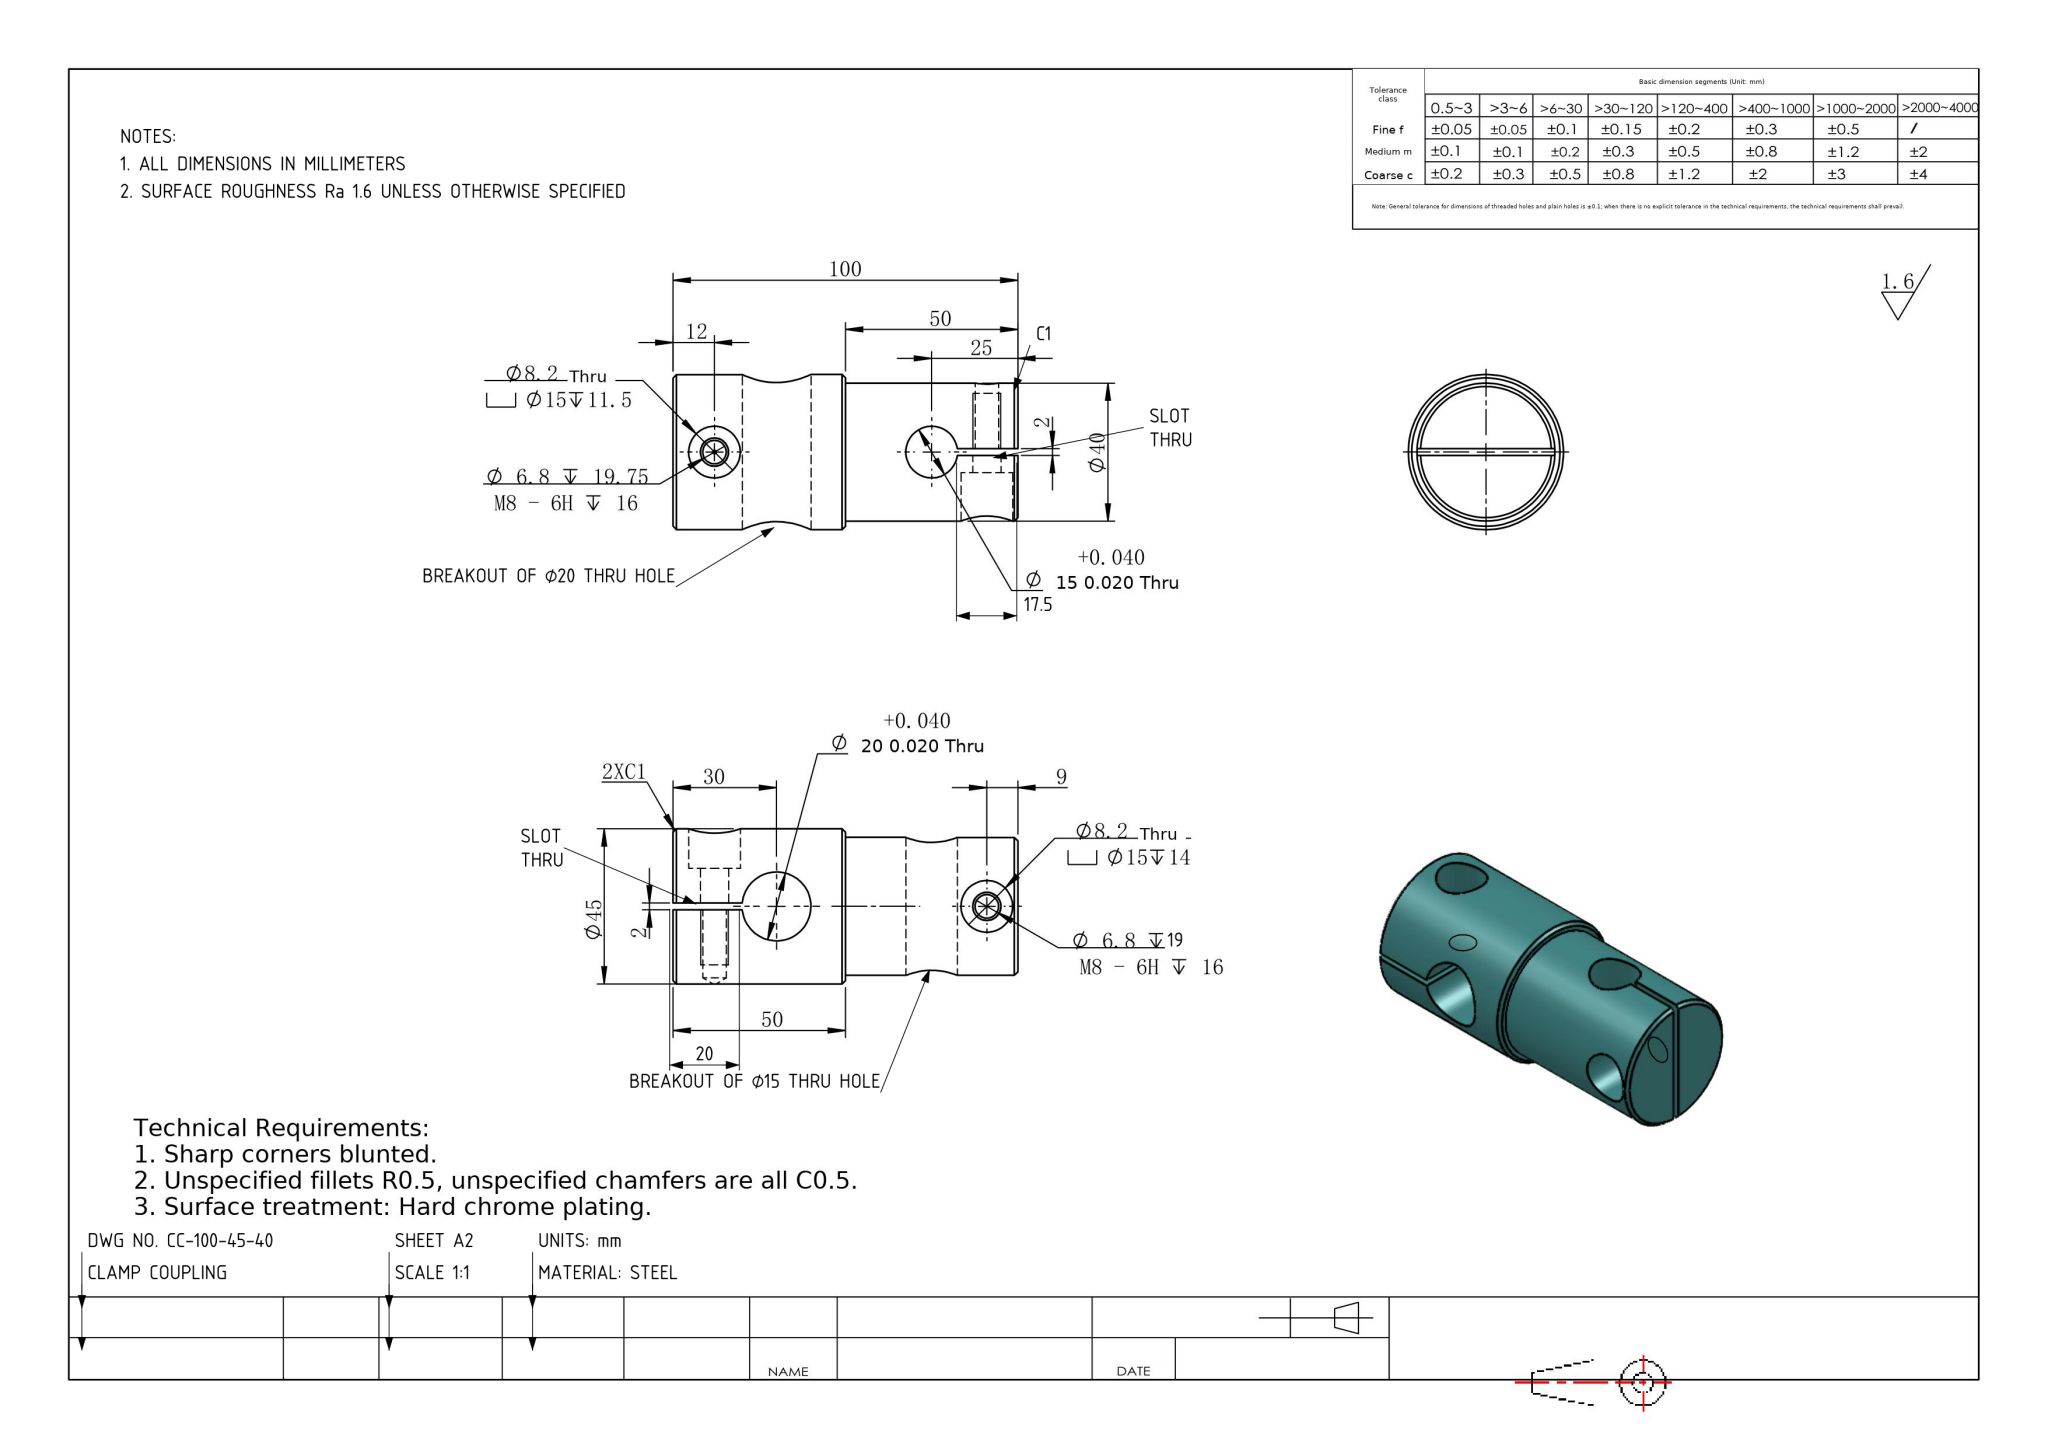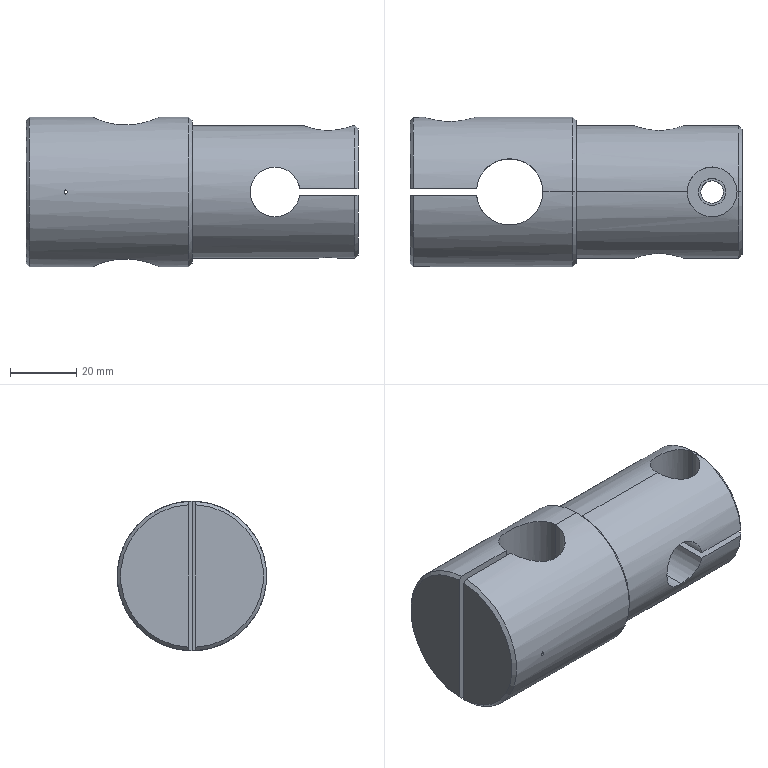Part | NX | mm | 1 solid | 41 faces | box 100 x 45 x 45 mm | volume 111624 mm3 | cylinder 21 | plane 11 | cone 9 | commonest cylinder face diameters 15 x7 8.2 x4 6.8 x4 20 x2 40 x2 45 x2